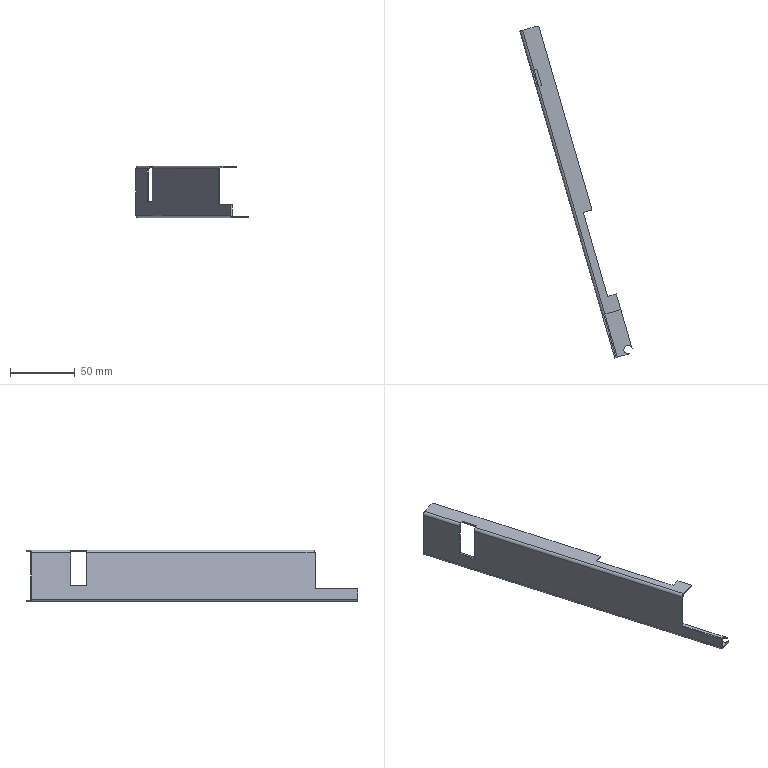Component | SolidWorks | LeftDoorAssembly-1_EndCap2-1 | 1 solid | 39 faces | volume 17430 mm3 | plane 30 | cylinder 9 | commonest cylinder face diameters 2 x5 4.4 x3 6.5 x1